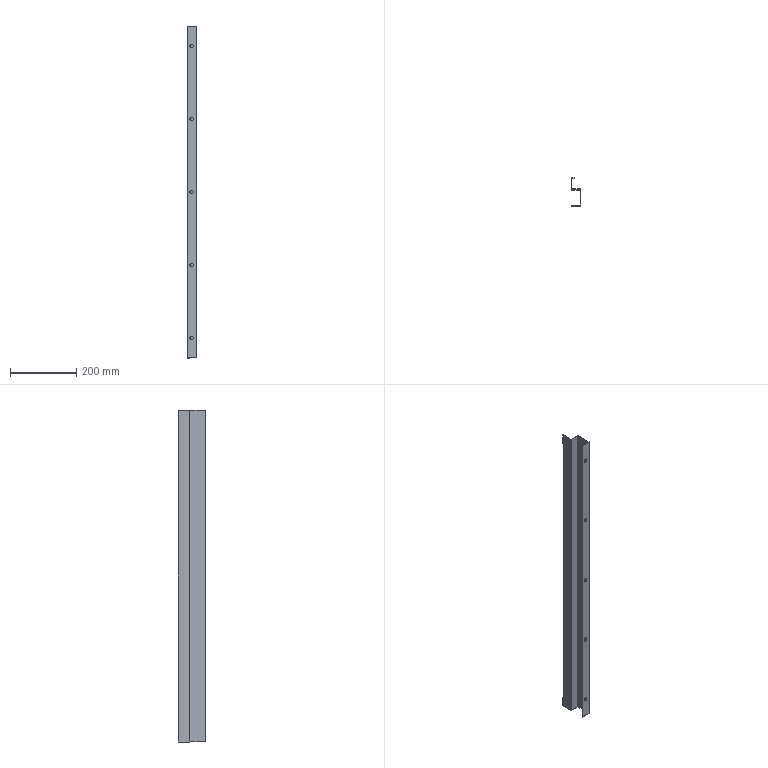Component | SolidWorks | SideLowerCrossbeam-1 | 1 solid | 52 faces | volume 219564 mm3 | plane 34 | cylinder 18 | commonest cylinder face diameters 11 x10 3.4 x4 0.4 x4